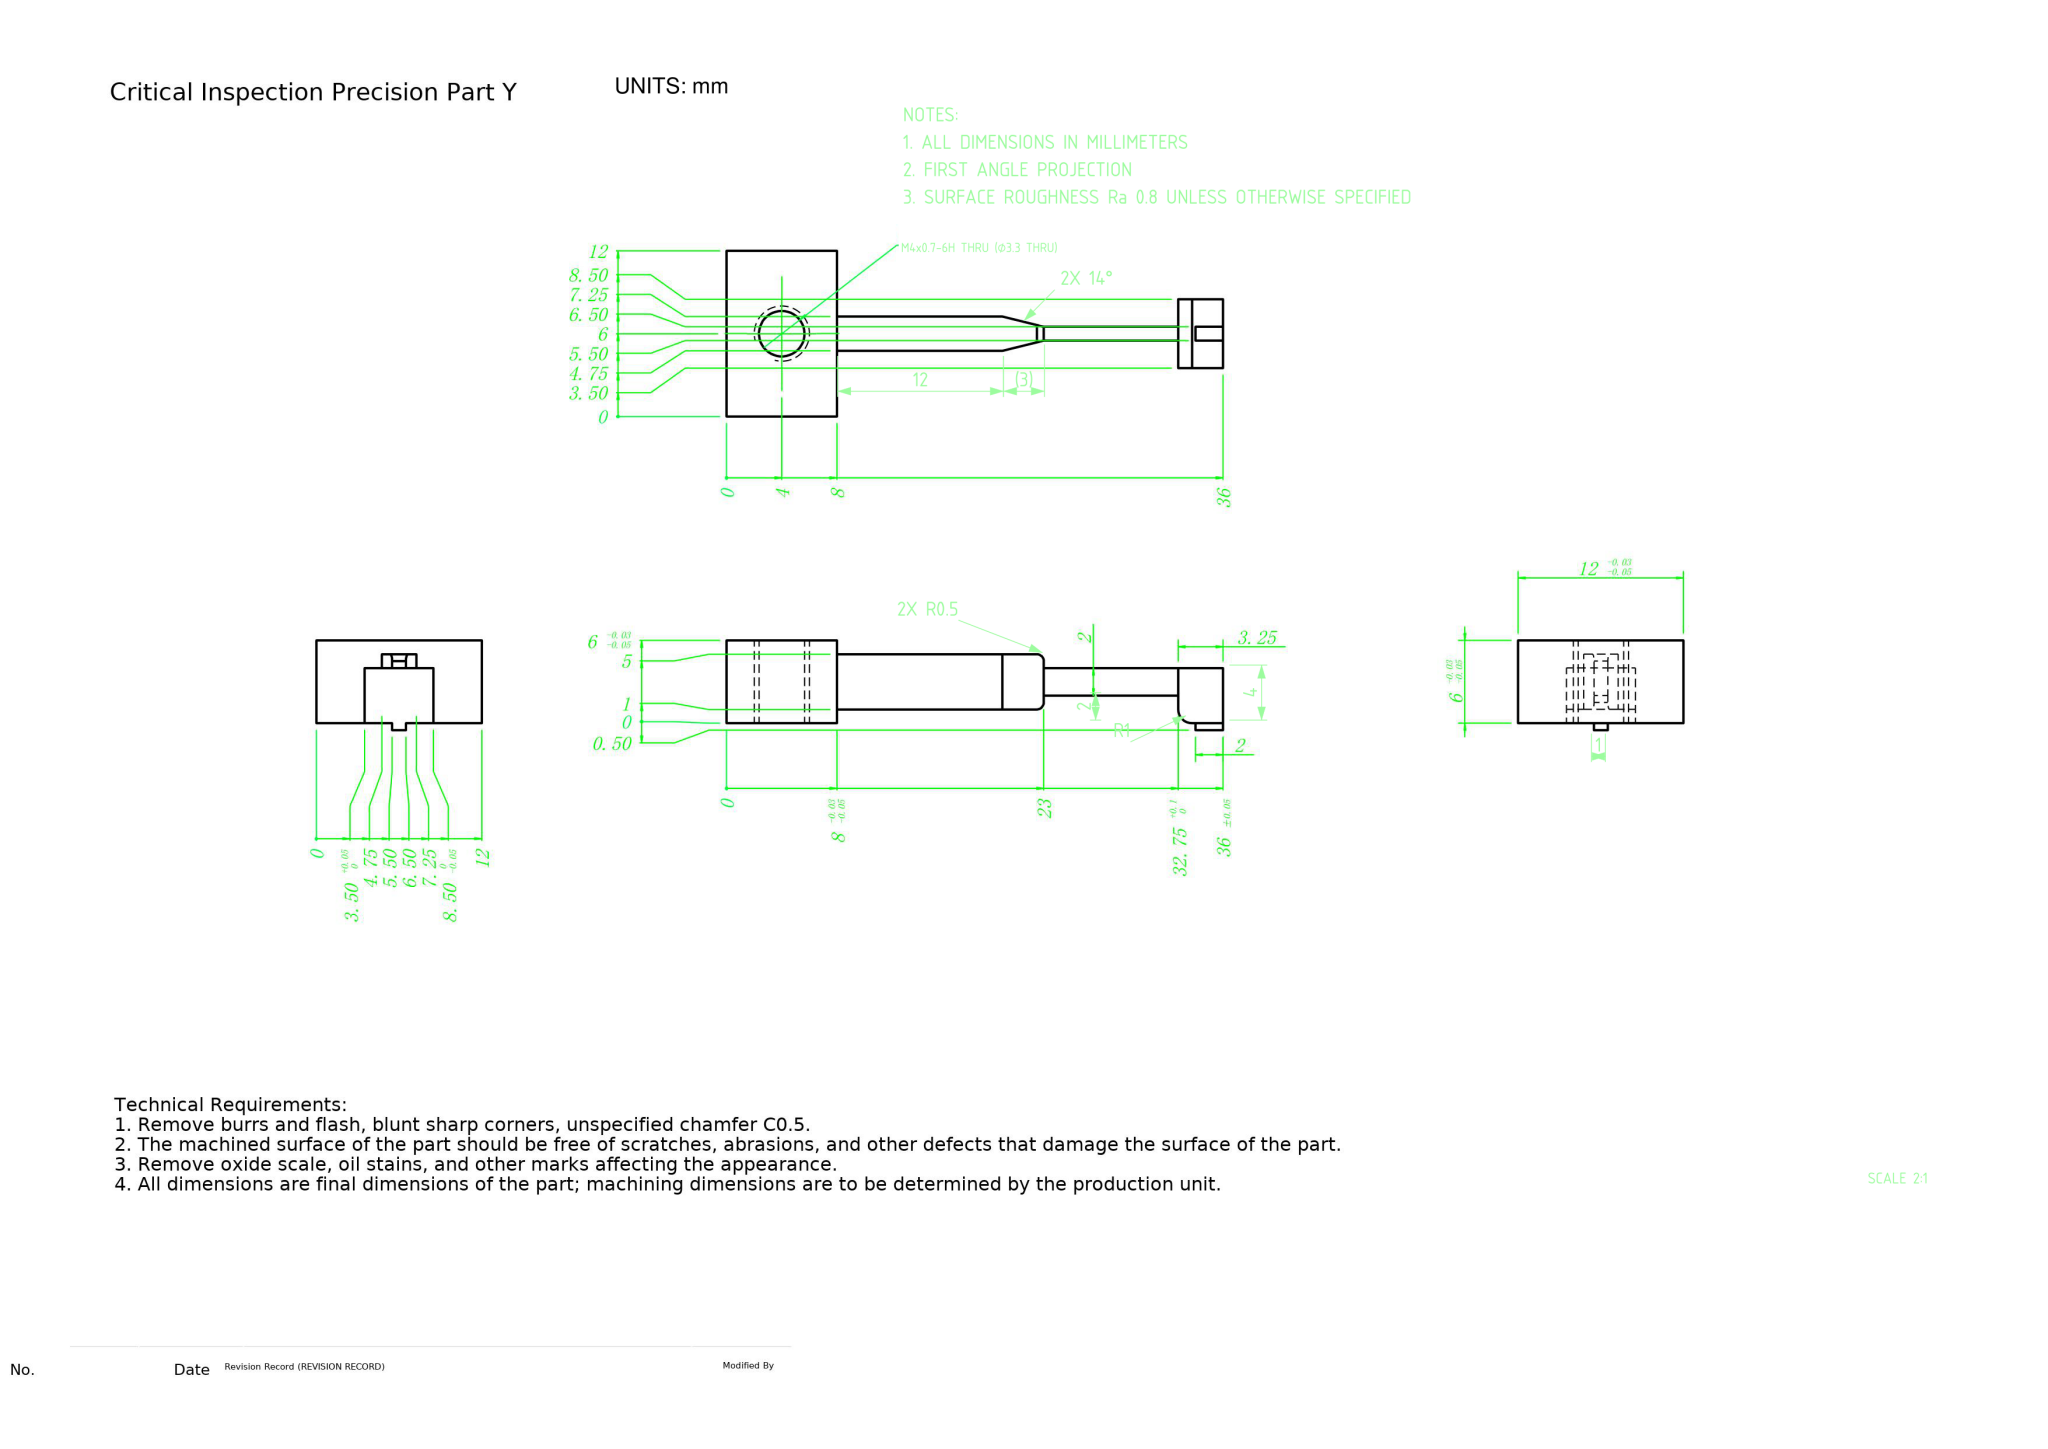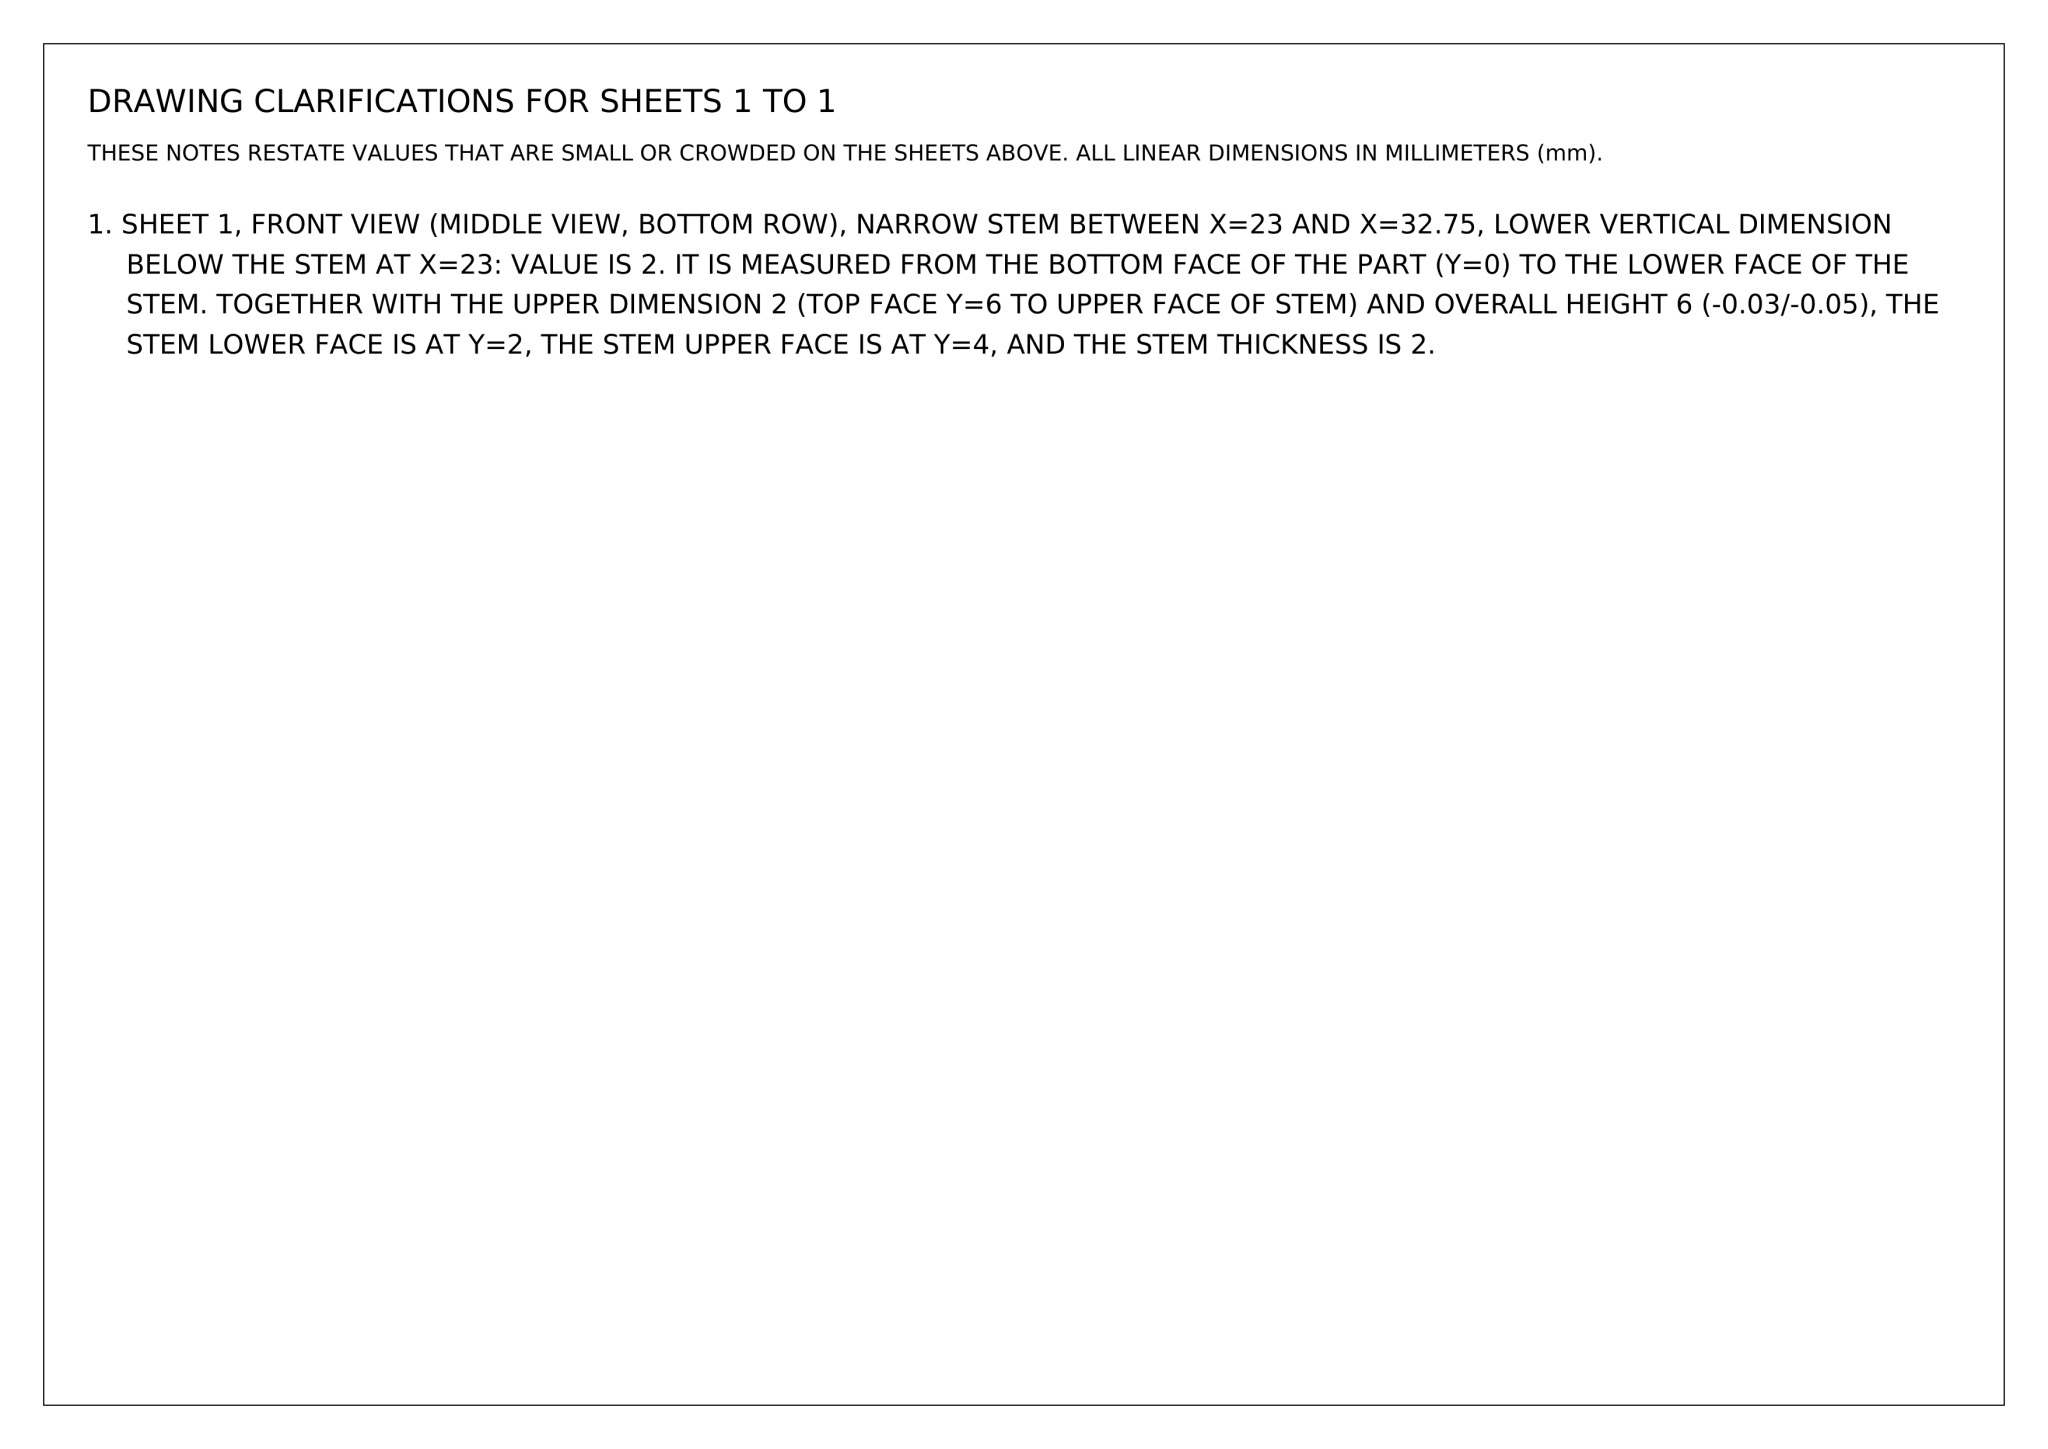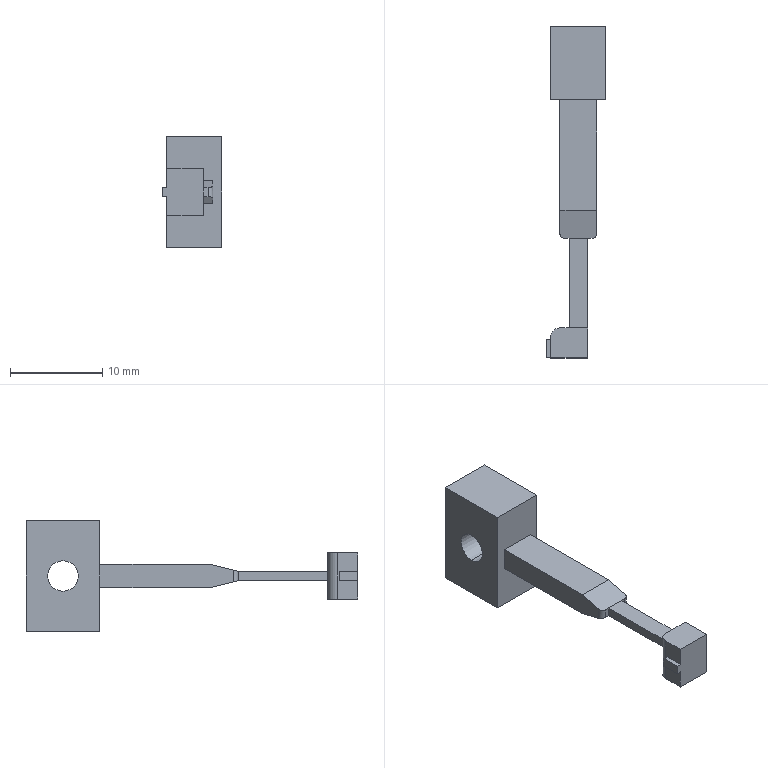Part | NX | mm | 1 solid | 32 faces | box 6.5 x 36 x 12 mm | volume 750 mm3 | plane 27 | cylinder 5 | commonest cylinder face diameters 3.3 x2 1 x2 2 x1